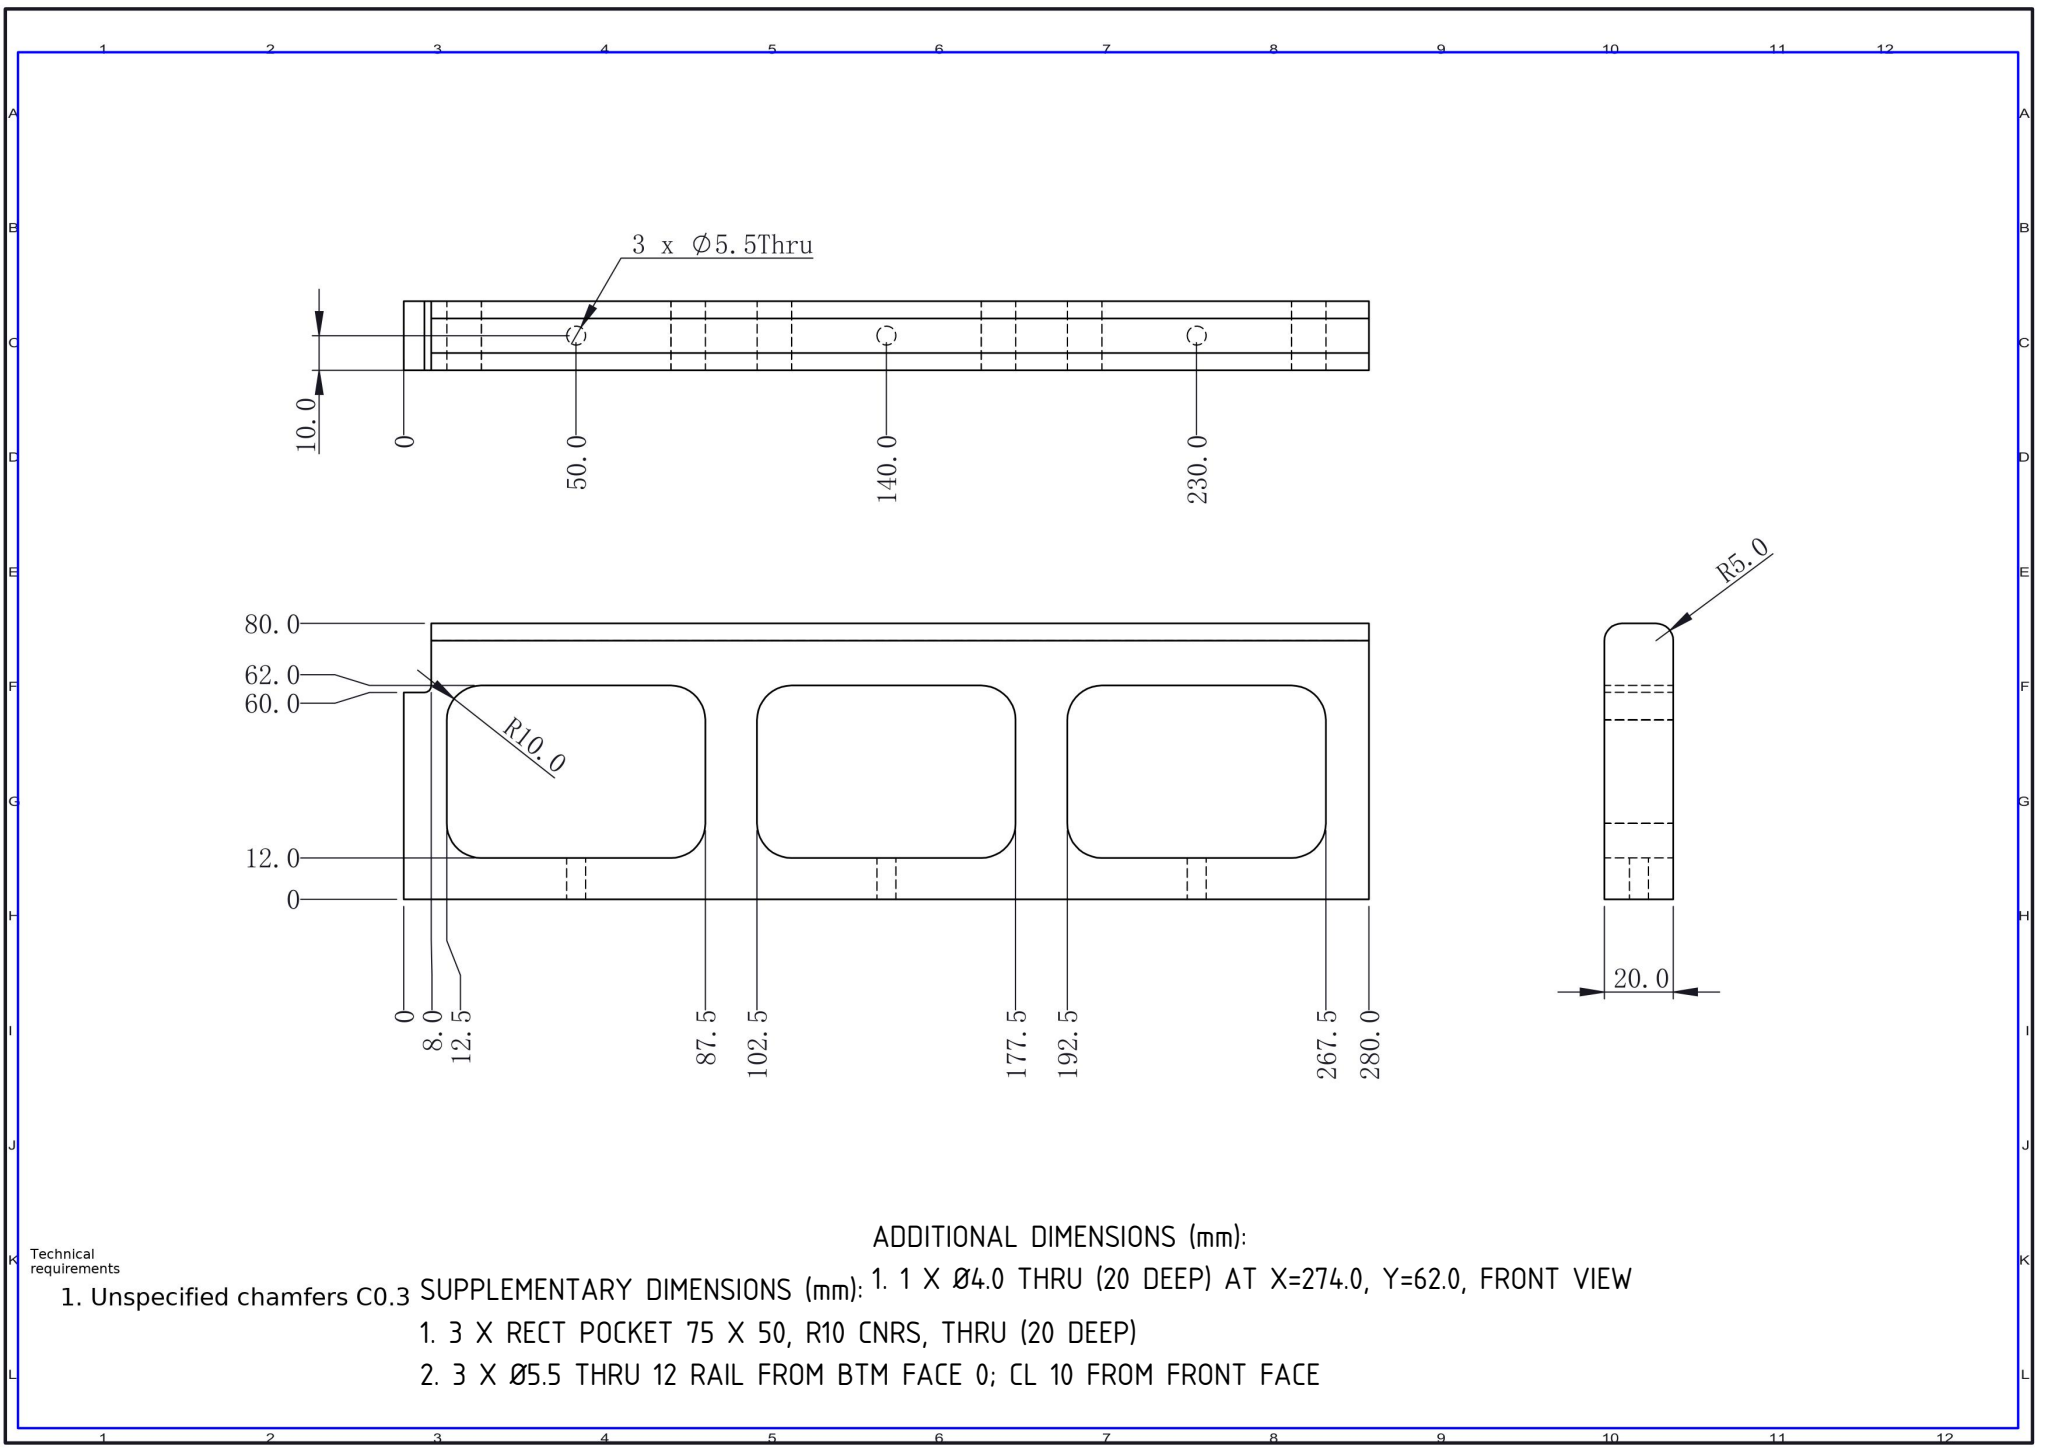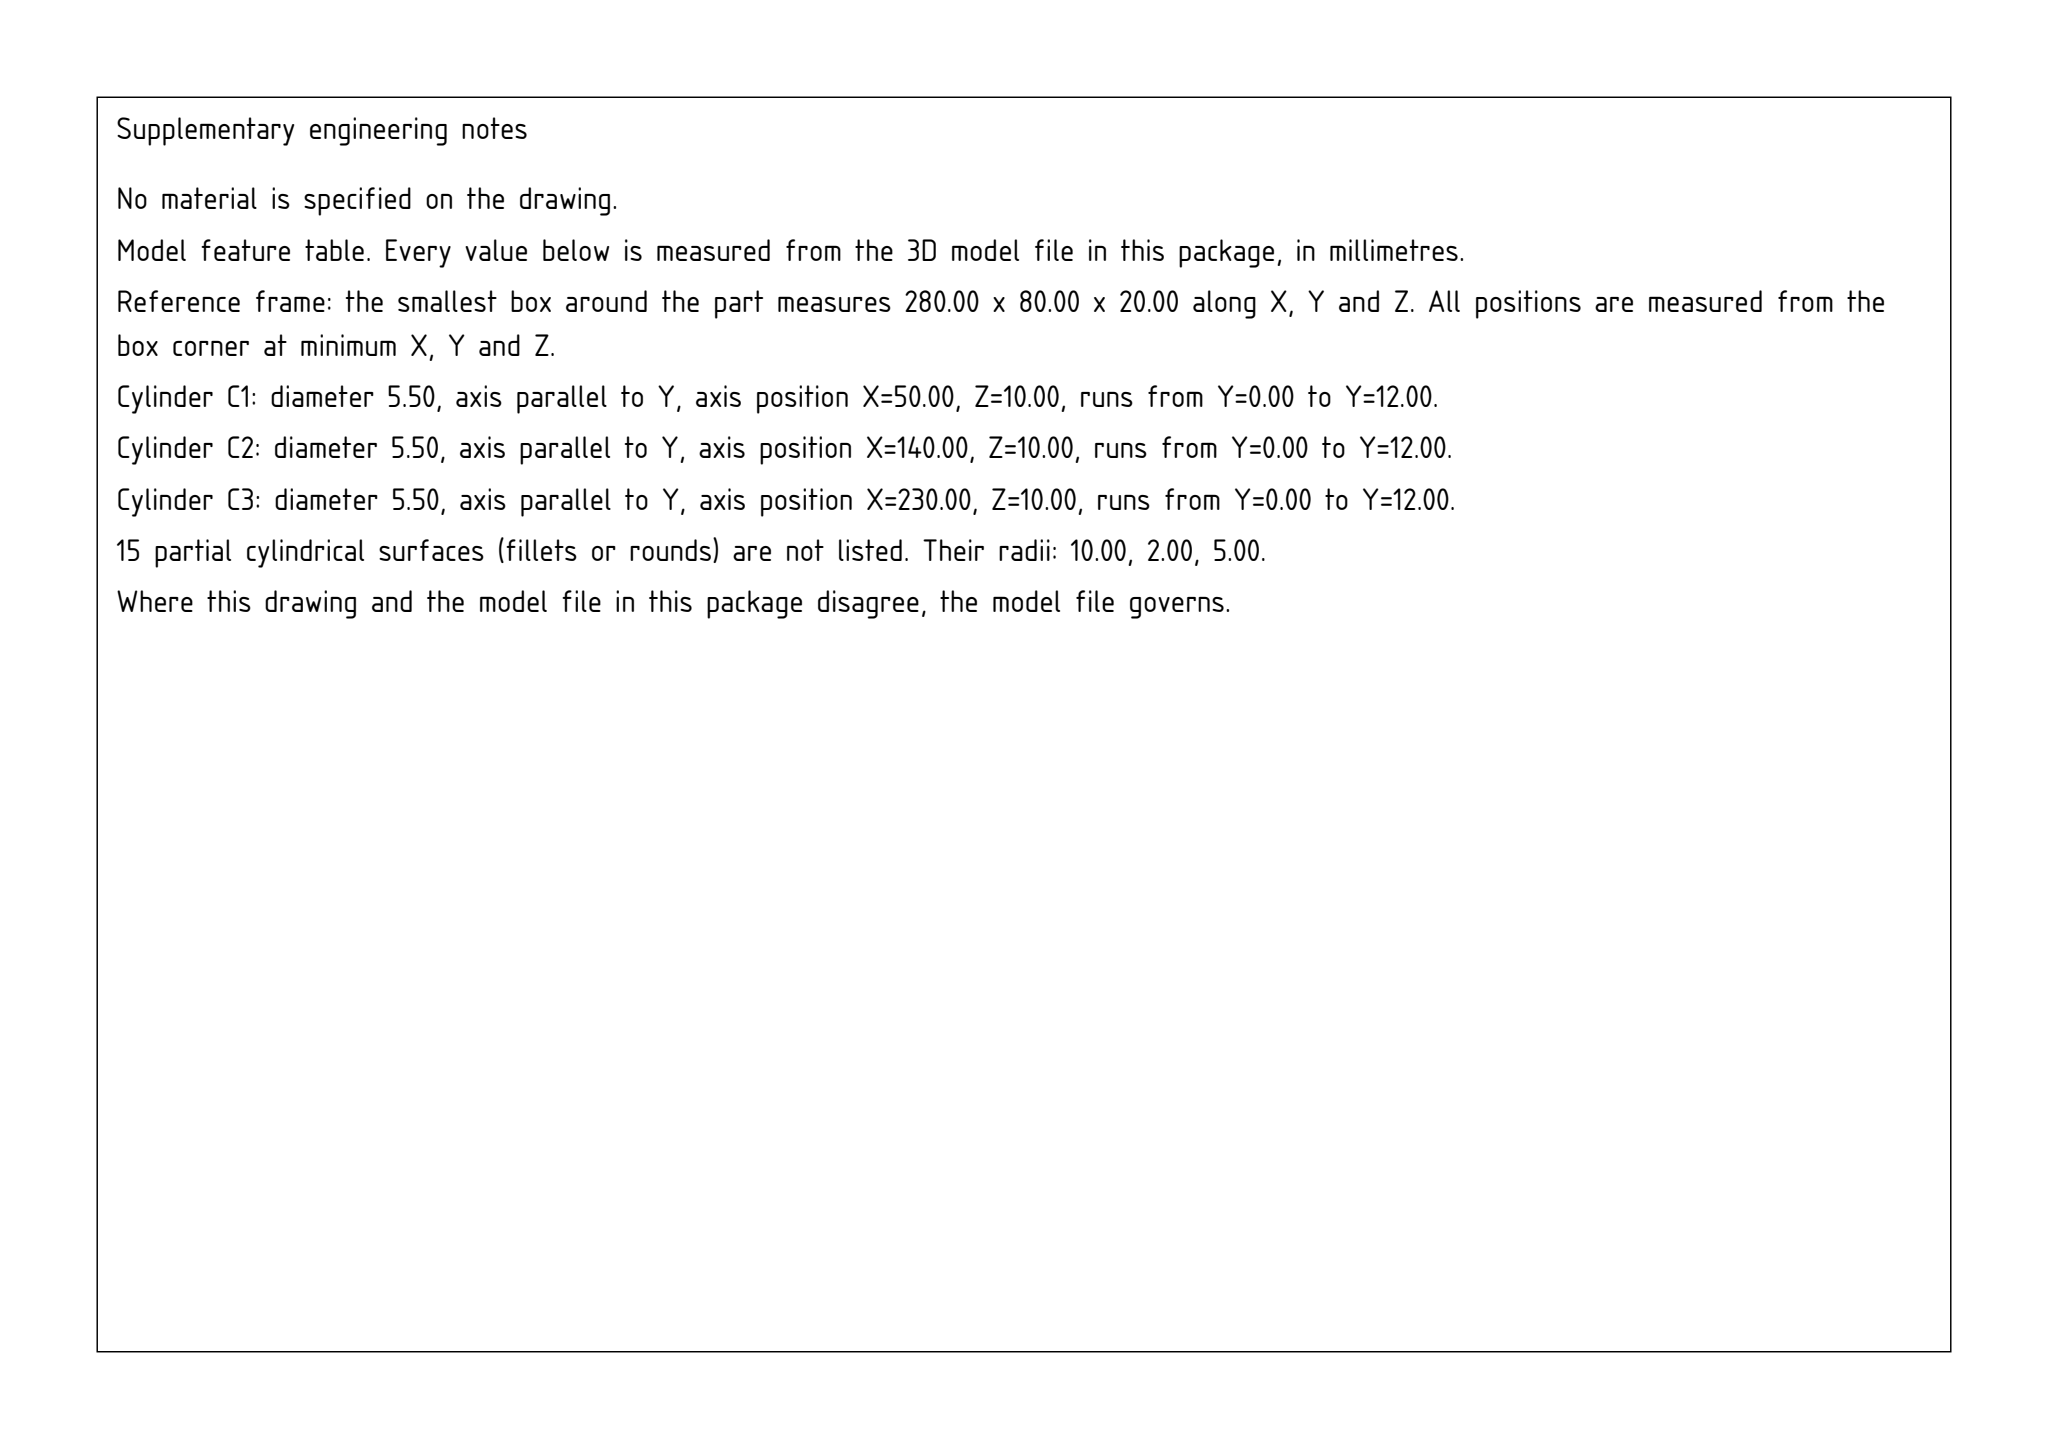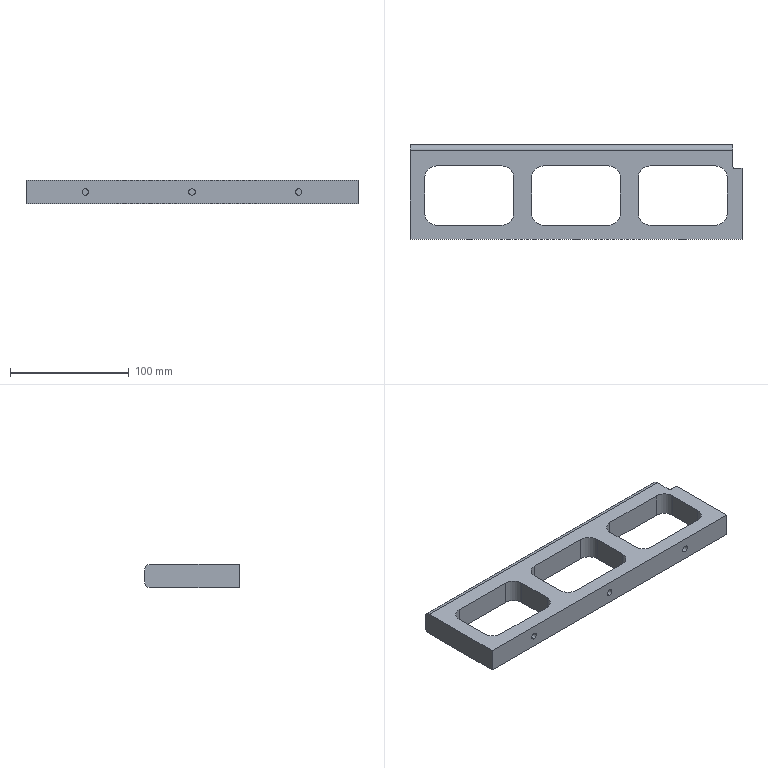Part | SolidWorks | mm | 1 solid | 41 faces | box 280 x 80 x 20 mm | volume 221194 mm3 | cylinder 21 | plane 20 | commonest cylinder face diameters 20 x12 5.5 x6 10 x2 4 x1
build123d program:
from build123d import *

# Parameters (mm, degrees)
SKETCH1_W                = 280
SKETCH1_H                = 80
BOSS_EXTRUDE1_DEPTH      = 20
FILLET1_R                = 5
CUT_EXTRUDE1_DEPTH       = 147.969
M5_CLEARANCE_HOLE1_D     = 5.5
M5_CLEARANCE_HOLE1_DEPTH = 12
CUT_EXTRUDE2_DEPTH       = 147.969
CUT_EXTRUDE2_DEPTH_BACK  = 147.969
SKETCH5_W                = 8
SKETCH5_H                = 20
FILLET2_R                = 2


with BuildPart() as part:
    # Sketch1 → Boss-Extrude1 (new body)
    with BuildSketch(Plane.XY):
        Rectangle(SKETCH1_W, SKETCH1_H)
    extrude(amount=BOSS_EXTRUDE1_DEPTH)

    # Fillet1
    fillet1_edges = [part.edges().sort_by_distance(p)[0] for p in [
        (0, 40, 0),
        (0, 40, 20),
    ]]
    fillet(fillet1_edges, radius=FILLET1_R)

    # Sketch2 → Cut-Extrude1 (cut, through all)
    with BuildSketch(Plane.XY.offset(20)):
        with BuildLine():
            Line((-117.5, -28), (-62.5, -28))
            ThreePointArc((-62.5, -28), (-55.429, -25.071), (-52.5, -18))
            Line((-52.5, -18), (-52.5, 12))
            ThreePointArc((-52.5, 12), (-55.429, 19.071), (-62.5, 22))
            Line((-62.5, 22), (-117.5, 22))
            ThreePointArc((-117.5, 22), (-124.571, 19.071), (-127.5, 12))
            Line((-127.5, 12), (-127.5, -18))
            ThreePointArc((-127.5, -18), (-124.571, -25.071), (-117.5, -28))
        make_face()
        with BuildLine():
            Line((-27.5, -28), (27.5, -28))
            ThreePointArc((27.5, -28), (34.571, -25.071), (37.5, -18))
            Line((37.5, -18), (37.5, 12))
            ThreePointArc((37.5, 12), (34.571, 19.071), (27.5, 22))
            Line((27.5, 22), (-27.5, 22))
            ThreePointArc((-27.5, 22), (-34.571, 19.071), (-37.5, 12))
            Line((-37.5, 12), (-37.5, -18))
            ThreePointArc((-37.5, -18), (-34.571, -25.071), (-27.5, -28))
        make_face()
        with BuildLine():
            Line((62.5, -28), (117.5, -28))
            ThreePointArc((117.5, -28), (124.571, -25.071), (127.5, -18))
            Line((127.5, -18), (127.5, 12))
            ThreePointArc((127.5, 12), (124.571, 19.071), (117.5, 22))
            Line((117.5, 22), (62.5, 22))
            ThreePointArc((62.5, 22), (55.429, 19.071), (52.5, 12))
            Line((52.5, 12), (52.5, -18))
            ThreePointArc((52.5, -18), (55.429, -25.071), (62.5, -28))
        make_face()
    extrude(amount=-CUT_EXTRUDE1_DEPTH, mode=Mode.SUBTRACT)

    # M5 Clearance Hole1
    with Locations(Plane(origin=(0, -40, 0), x_dir=(-1, 0, 0), z_dir=(0, -1, 0))):
        with Locations((90, -10), (0, -10), (-90, -10)):
            Hole(M5_CLEARANCE_HOLE1_D / 2, depth=M5_CLEARANCE_HOLE1_DEPTH)

    # Sketch5 → Cut-Extrude2 (cut, two sides: drawn at the far end of the back side and taken through both)
    with BuildSketch(Plane(origin=(0, 0, 0), x_dir=(-1, 0, 0), z_dir=(0, 0, -1)).offset(-CUT_EXTRUDE2_DEPTH_BACK)):
        with Locations((-136, 30)):
            Rectangle(SKETCH5_W, SKETCH5_H)
    extrude(amount=CUT_EXTRUDE2_DEPTH + CUT_EXTRUDE2_DEPTH_BACK, mode=Mode.SUBTRACT)

    # Fillet2
    fillet2_edges = [part.edges().sort_by_distance(p)[0] for p in [
        (132, 20, 10),
    ]]
    fillet(fillet2_edges, radius=FILLET2_R)


solid = part.part